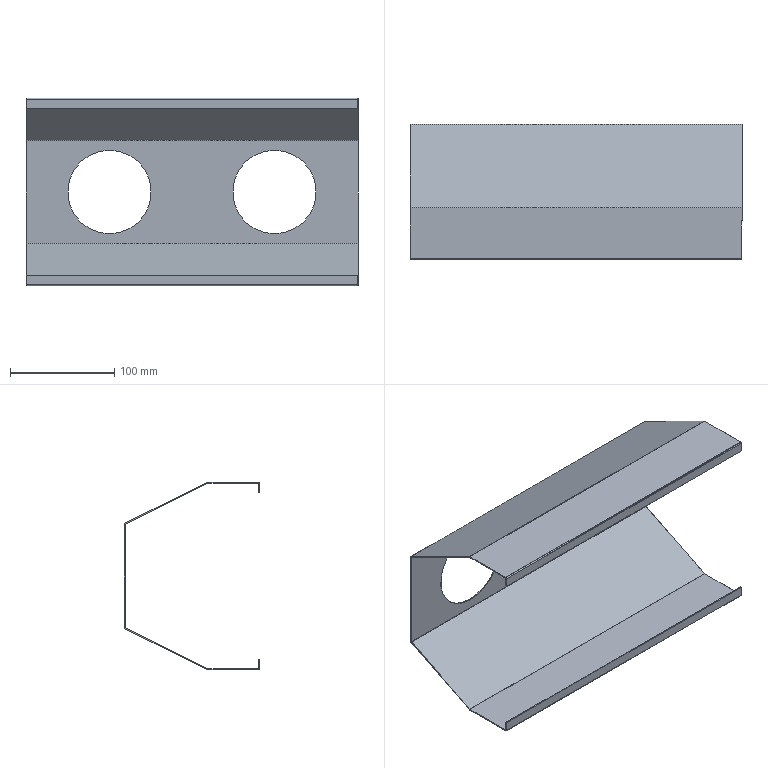Component | SolidWorks | LightBox-1_LightBox1-1 | 1 solid | 58 faces | volume 115397 mm3 | plane 42 | cylinder 16 | commonest cylinder face diameters 2.2 x6 0.2 x6 80 x4